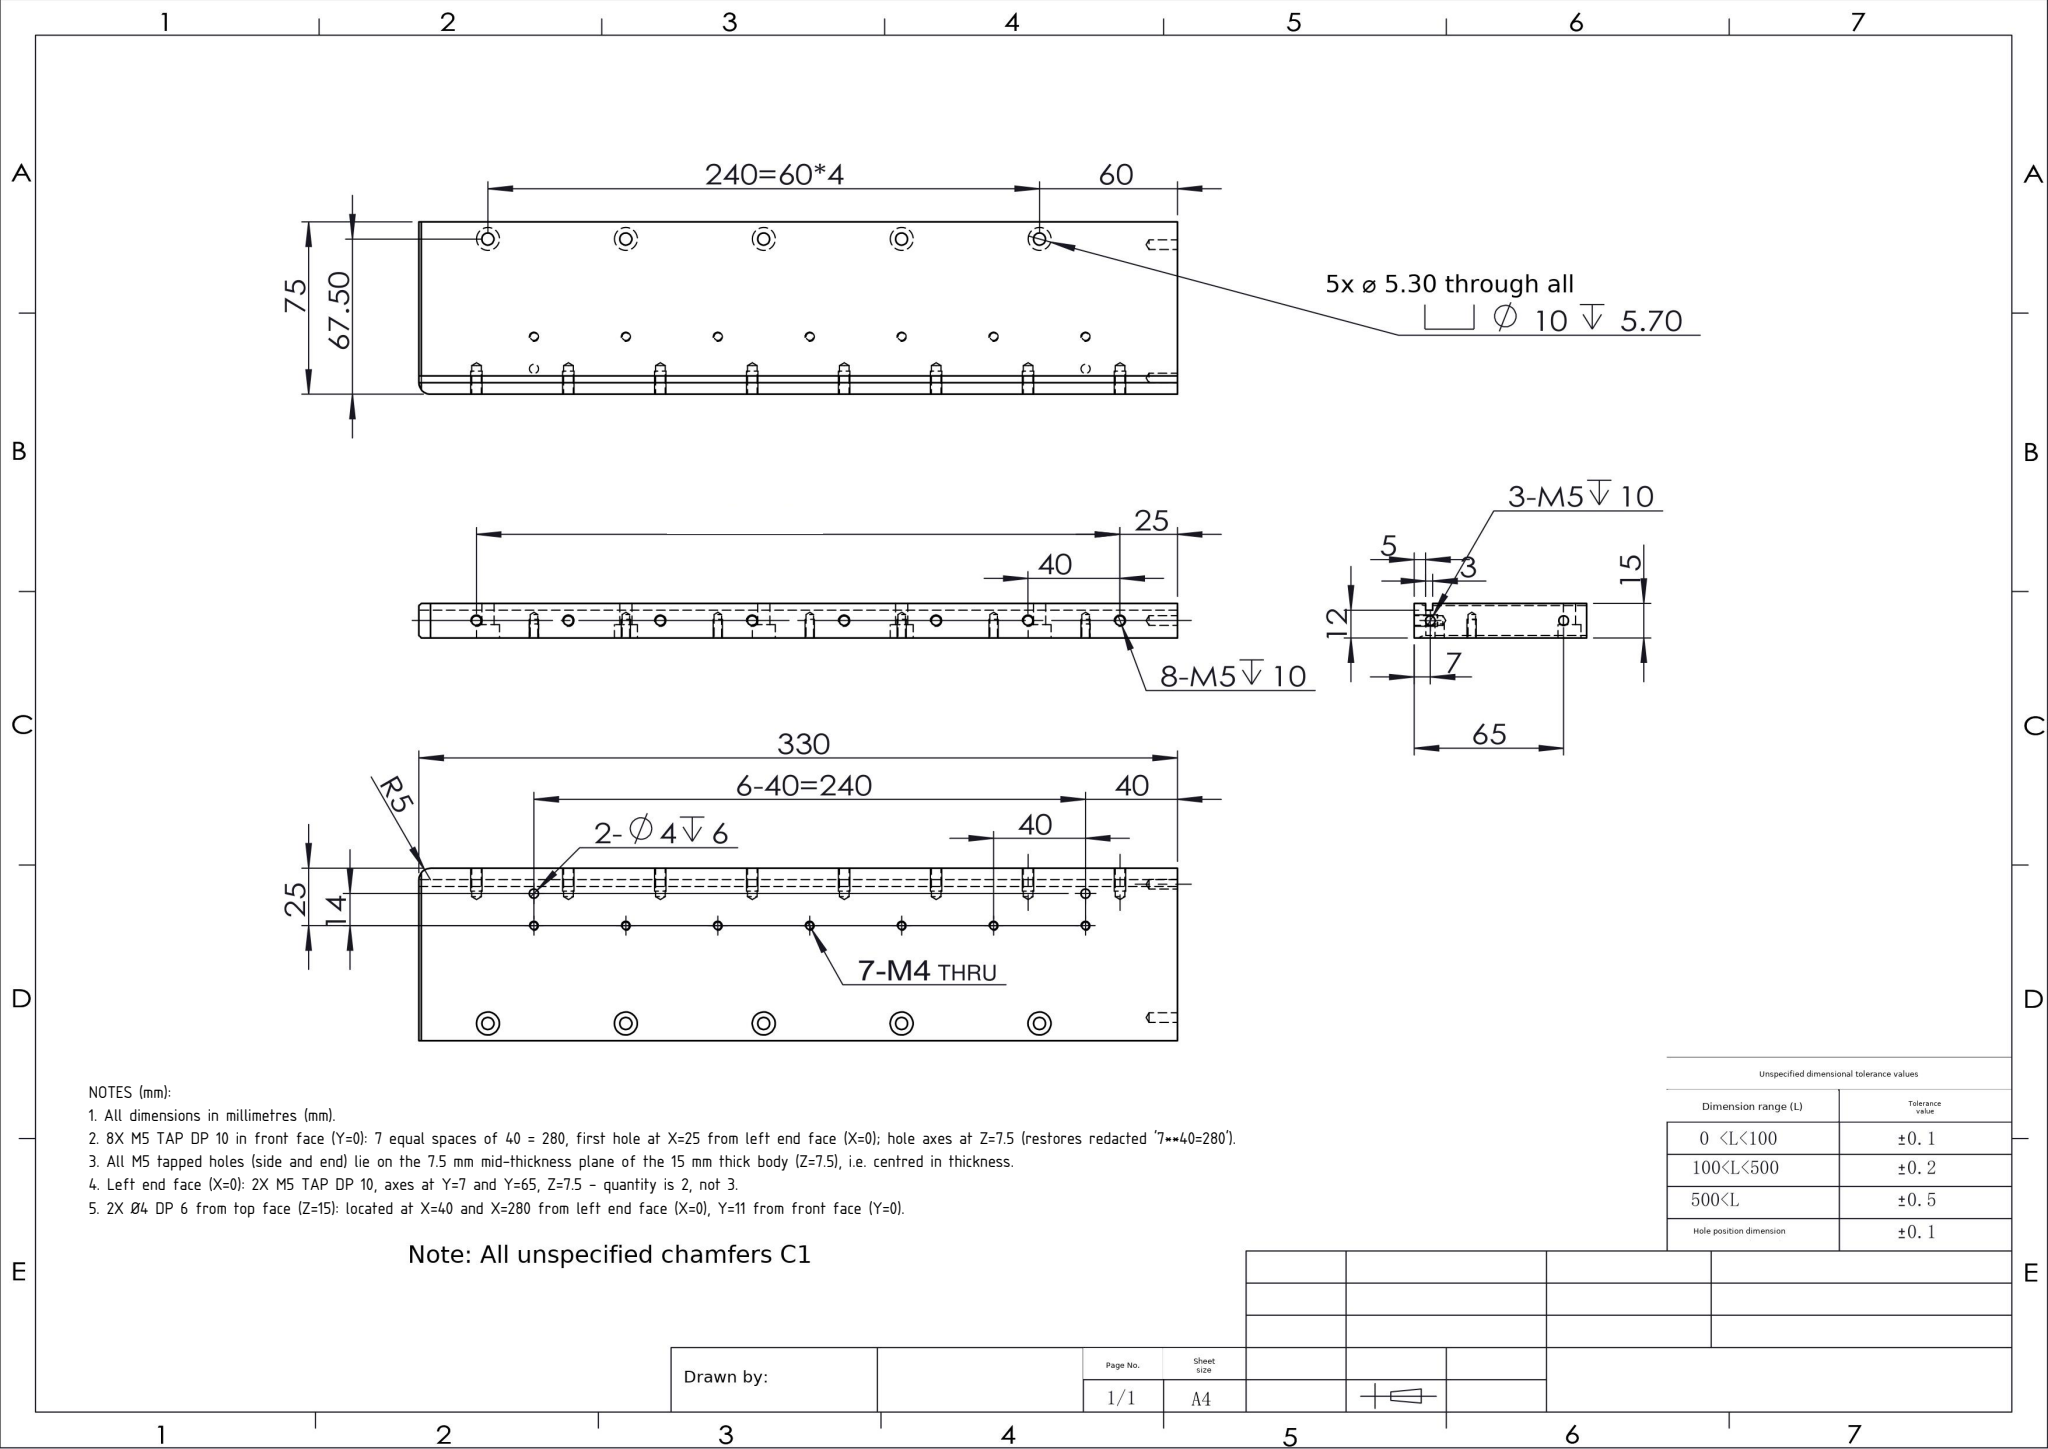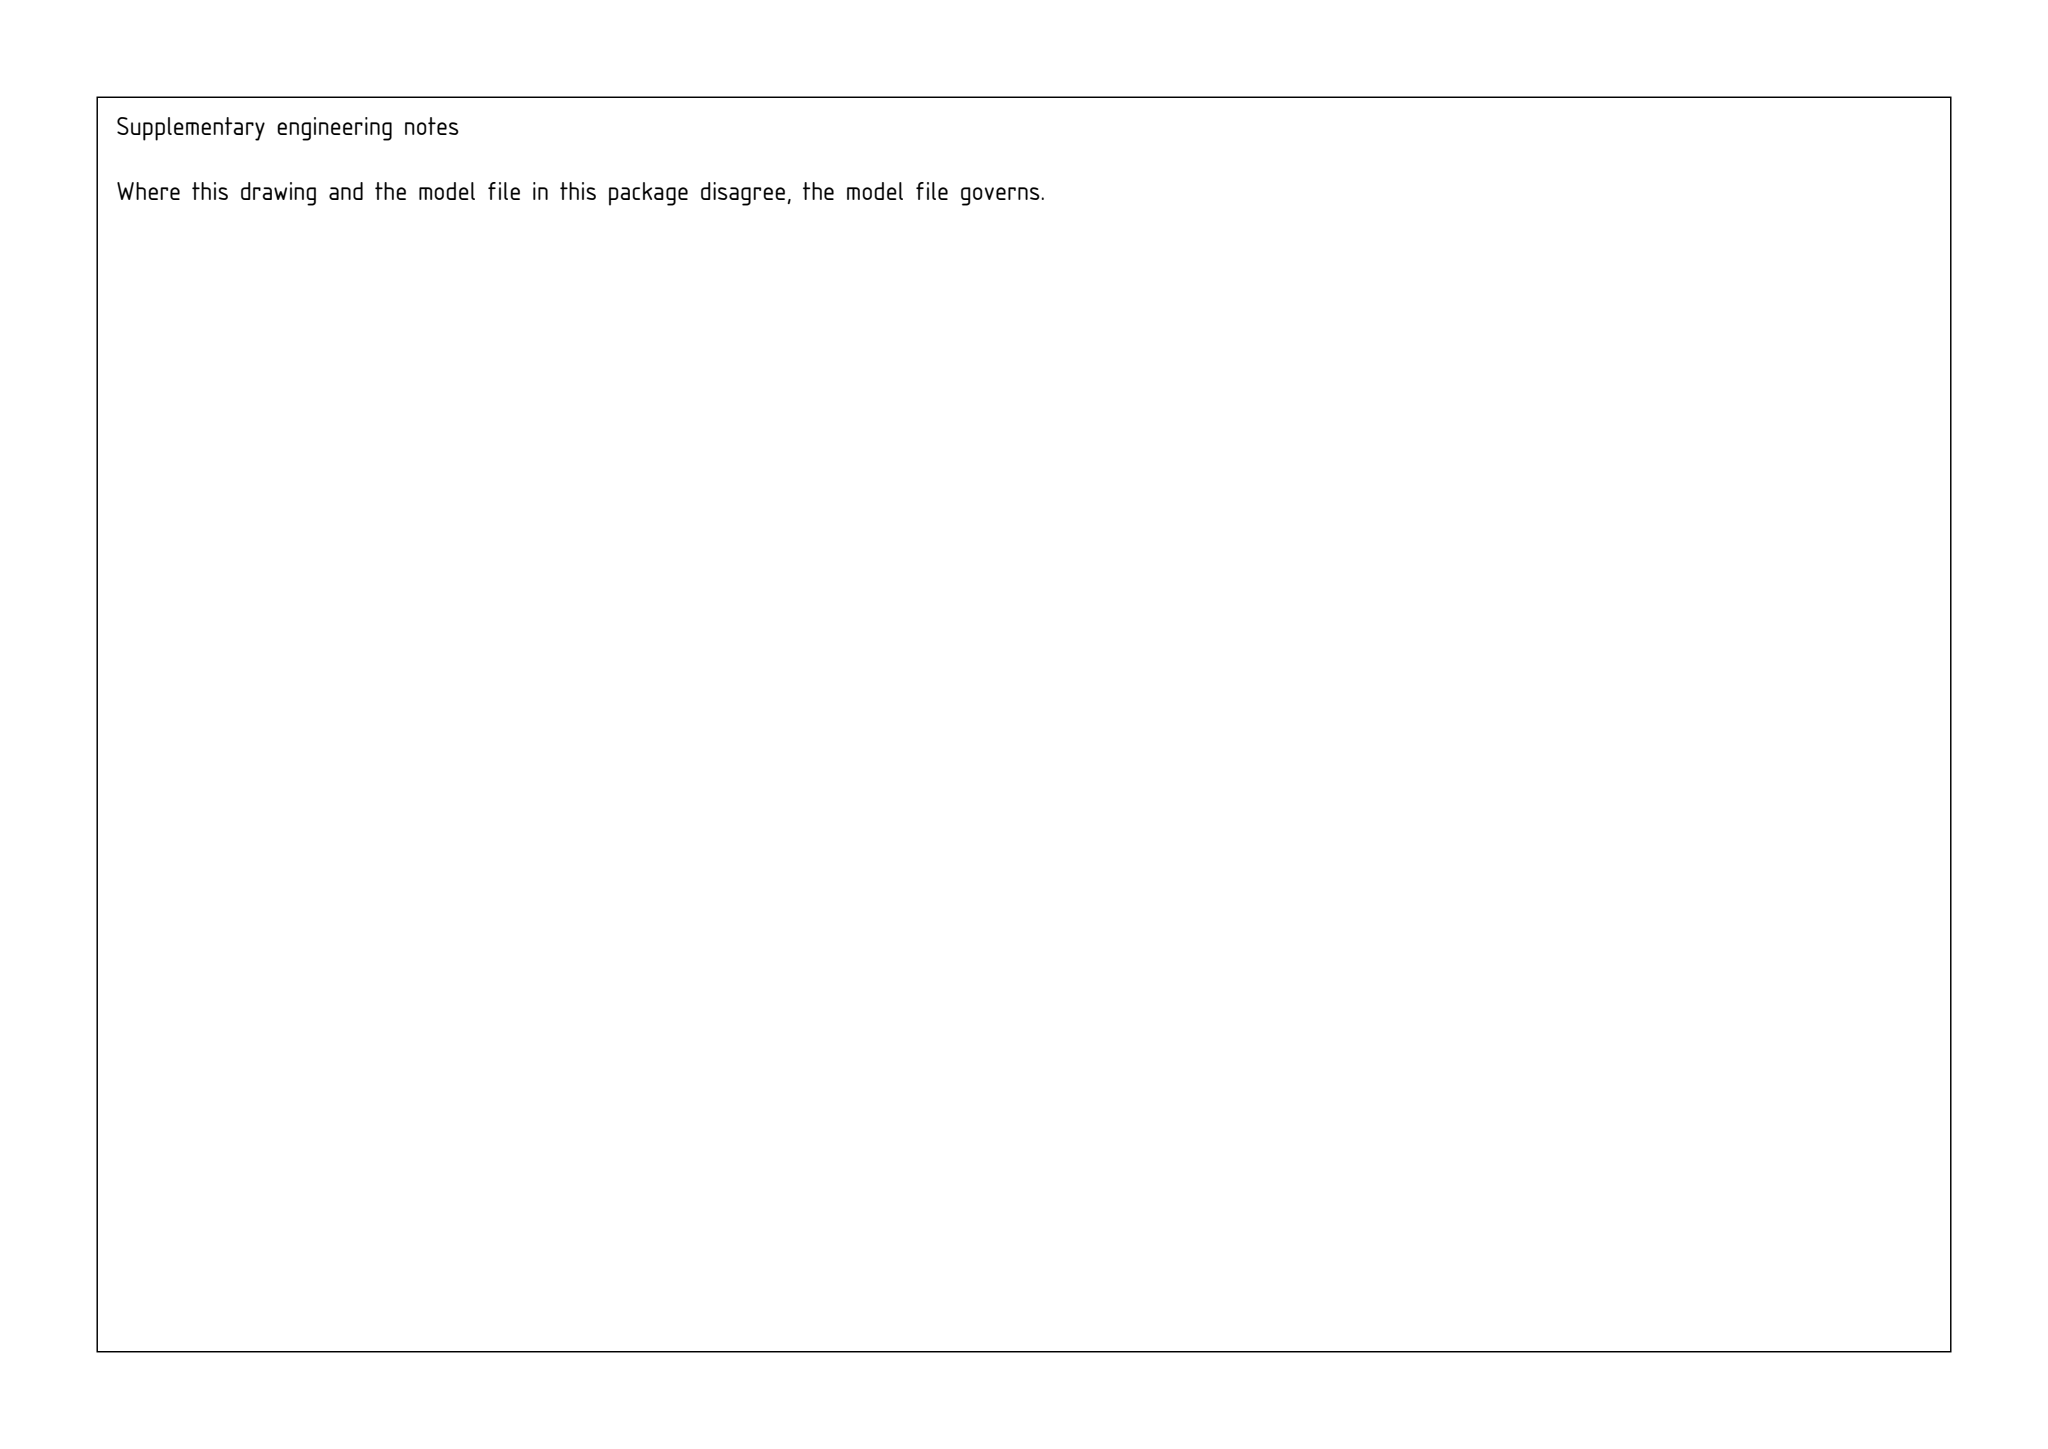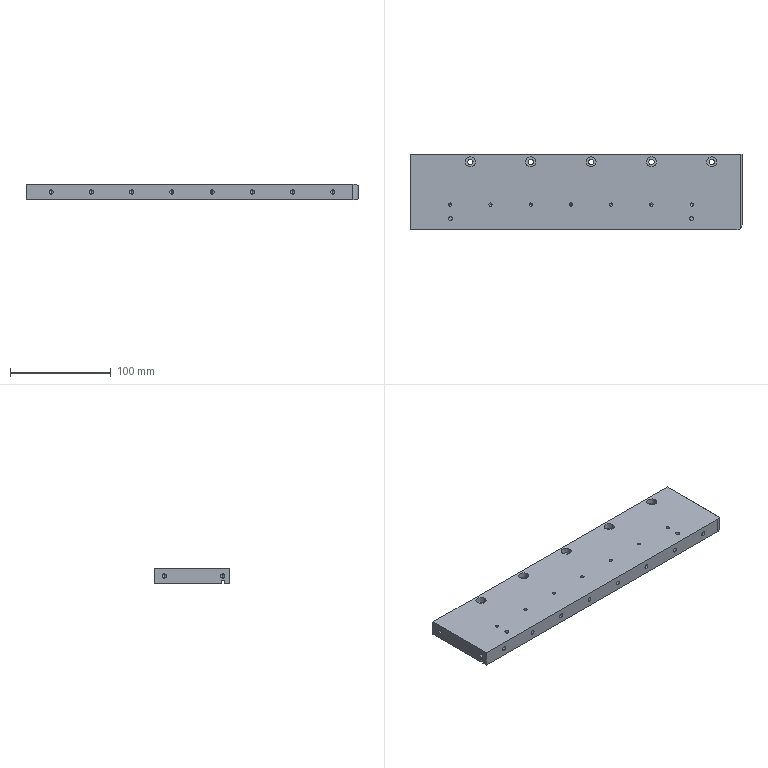Part | SolidWorks | mm | 1 solid | 113 faces | box 330 x 75 x 15 mm | volume 362314 mm3 | cylinder 59 | cone 34 | plane 20 | commonest cylinder face diameters 4.2 x20 3.3 x14 10 x11 5.3 x10 4 x4
Drawing notes:
All dimensions in millimetres (mm). | from the solid: STEP model facts stated in mm; bbox_xyz = 330.0 x 75.0 x 15.0
8X M5 TAP DP 10 in front face (Y=0): 7 equal spaces of 40 = 280, first hole at X=25 from left end face (X=0); hole axes at Z=7.5 (restores redacted '7**40=280'). | from the solid: cylinders: 8x hole/bore dia 4.2, axis y, at x = 25,65,105,145,185,225,265,305, z = 7.5, from 0 to 12.4
All M5 tapped holes (side and end) lie on the 7.5 mm mid-thickness plane of the 15 mm thick body (Z=7.5), i.e. centred in thickness. | from the solid: cylinders: all dia 4.2 bores (axis x and axis y) have axis_pos z = 7.5; bbox z extent 0-15
Left end face (X=0): 2X M5 TAP DP 10, axes at Y=7 and Y=65, Z=7.5 - quantity is 2, not 3. | from the solid: cylinders: only two dia 4.2 bores with axis x, at [y=7.0, z=7.5] and [y=65.0, z=7.5], from 0 to 12.4
2X Ø4 DP 6 from top face (Z=15): located at X=40 and X=280 from left end face (X=0), Y=11 from front face (Y=0). | from the solid: cylinders: hole/bore dia 4.0, axis z, at [40.0, 11.0] and [280.0, 11.0], from 9.0 to 15.0
build123d program:
from build123d import *

# Parameters (mm, degrees)
SKETCH1_W                                            = 330
SKETCH1_H                                            = 100
BOSS_EXTRUDE1_DEPTH                                  = 15
FILLET1_R                                            = 10
CUT_EXTRUDE2_DEPTH                                   = 0.1
CHAMFER1_SIZE                                        = 1
CHAMFER2_SIZE                                        = 1
CUT_EXTRUDE5_START                                   = -12
SKETCH14_W                                           = 717.936
SKETCH14_H                                           = 3
CUT_EXTRUDE5_DEPTH                                   = 3
FILLET5_R                                            = 5
LPATTERN5_COUNT                                      = 8
LPATTERN5_PITCH                                      = 40
M5_TAPPED_HOLE2_D                                    = 4.2
M5_TAPPED_HOLE2_DEPTH                                = 12.4
M5_TAPPED_HOLE2_TIP                                  = 1.262
HOLE_SIZE_ACCORDING_TO_THE_TYPE_OF_HEXAG_D           = 5.3
HOLE_SIZE_ACCORDING_TO_THE_TYPE_OF_HEXAG_CBORE_D     = 10
HOLE_SIZE_ACCORDING_TO_THE_TYPE_OF_HEXAG_CBORE_DEPTH = 5.7
LPATTERN6_COUNT                                      = 5
LPATTERN6_PITCH                                      = 60
LPATTERN7_COUNT                                      = 7
LPATTERN7_PITCH                                      = 40
SKETCH27_R                                           = 2
CUT_EXTRUDE6_DEPTH                                   = 6
SKETCH28_W                                           = 438.351
SKETCH28_H                                           = 72.886
CUT_EXTRUDE7_DEPTH                                   = 346.145
HOLE_SIZE_ACCORDING_TO_THE_TYPE_OF_H_2_D             = 5.3
HOLE_SIZE_ACCORDING_TO_THE_TYPE_OF_H_2_CBORE_D       = 10
HOLE_SIZE_ACCORDING_TO_THE_TYPE_OF_H_2_CBORE_DEPTH   = 5.7


with BuildPart() as part:
    # Sketch1 → Boss-Extrude1 (new body)
    with BuildSketch(Plane.XY):
        with Locations((165, -50)):
            Rectangle(SKETCH1_W, SKETCH1_H)
    extrude(amount=BOSS_EXTRUDE1_DEPTH)

    # Fillet1
    fillet1_edges = [part.edges().sort_by_distance(p)[0] for p in [
        (330, 0, 7.5),
    ]]
    fillet(fillet1_edges, radius=FILLET1_R)

    # Sketch2 → Cut-Extrude2 (cut)
    with BuildSketch(Plane.XY.offset(15)):
        with BuildLine():
            Line((63.85, -16.145), (63.165, -16.311))
            Line((63.165, -16.311), (63.004, -17.061))
            Line((63.004, -17.061), (62.928, -17.444))
            Line((62.928, -17.444), (62.898, -17.565))
            add(Edge.make_bspline(
                [(62.898, -17.565), (62.895, -17.573), (62.89, -17.588), (62.88, -17.605), (62.869, -17.613), (62.856, -17.615), (62.847, -17.604), (62.842, -17.591), (62.84, -17.571), (62.835, -17.545), (62.833, -17.508), (62.829, -17.48), (62.827, -17.464)],
                knots=[0, 0, 0, 0, 1.227, 2.069, 2.596, 3.064, 3.56, 4.322, 5.03, 6.209, 7.852, 10, 10, 10, 10], degree=3))
            Line((62.827, -17.464), (62.803, -17.253))
            add(Edge.make_bspline(
                [(62.803, -17.253), (62.801, -17.235), (62.798, -17.204), (62.796, -17.163), (62.796, -17.134), (62.797, -17.109), (62.804, -17.086), (62.813, -17.069), (62.818, -17.061)],
                knots=[0, 0, 0, 0, 1.604, 2.861, 3.774, 4.323, 5.132, 6, 6, 6, 6], degree=3))
            Line((62.818, -17.061), (62.843, -17.016))
            add(Edge.make_bspline(
                [(62.843, -17.016), (62.848, -17.004), (62.861, -16.976), (62.878, -16.923), (62.895, -16.856), (62.913, -16.778), (62.93, -16.702), (62.944, -16.64), (62.955, -16.599), (62.962, -16.579), (62.964, -16.573)],
                knots=[0, 0, 0, 0, 0.6797, 1.623, 2.844, 4.336, 5.799, 6.891, 7.631, 8, 8, 8, 8], degree=3))
            Line((62.964, -16.573), (63.482, -14.172))
            Line((63.482, -14.172), (63.552, -14.172))
            Line((63.552, -14.172), (64.041, -16.331))
            Line((64.041, -16.331), (64.101, -16.583))
            add(Edge.make_bspline(
                [(64.101, -16.583), (64.107, -16.611), (64.118, -16.662), (64.135, -16.73), (64.148, -16.781), (64.158, -16.808), (64.162, -16.82)],
                knots=[0, 0, 0, 0, 1.426, 2.558, 3.42, 4, 4, 4, 4], degree=3))
            Line((64.162, -16.82), (64.197, -16.915))
            add(Edge.make_bspline(
                [(64.197, -16.915), (64.201, -16.929), (64.208, -16.954), (64.221, -16.988), (64.233, -17.014), (64.249, -17.036), (64.265, -17.053), (64.276, -17.07), (64.277, -17.086), (64.275, -17.1), (64.273, -17.119), (64.272, -17.142), (64.269, -17.174), (64.268, -17.199), (64.268, -17.213)],
                knots=[0, 0, 0, 0, 1.645, 2.997, 4.066, 4.893, 6.03, 6.671, 7.125, 7.802, 8.339, 9.24, 10.452, 12, 12, 12, 12], degree=3))
            Line((64.268, -17.213), (64.247, -17.439))
            Line((64.247, -17.439), (64.237, -17.524))
            add(Edge.make_bspline(
                [(64.237, -17.524), (64.236, -17.534), (64.236, -17.551), (64.231, -17.574), (64.229, -17.59), (64.223, -17.601), (64.212, -17.607), (64.198, -17.603), (64.187, -17.589), (64.184, -17.577), (64.182, -17.57)],
                knots=[0, 0, 0, 0, 1.663, 2.956, 3.874, 4.465, 5.131, 5.832, 6.736, 8, 8, 8, 8], degree=3))
            Line((64.182, -17.57), (64.147, -17.368))
            Line((64.147, -17.368), (63.85, -16.145))
        make_face()
        with BuildLine():
            Line((63.839, -16.069), (63.517, -14.655))
            Line((63.517, -14.655), (63.19, -16.135))
            add(Edge.make_bspline(
                [(63.19, -16.135), (63.218, -16.13), (63.267, -16.123), (63.336, -16.108), (63.4, -16.09), (63.458, -16.074), (63.505, -16.058), (63.536, -16.047), (63.56, -16.036), (63.572, -16.028), (63.578, -16.024)],
                knots=[0, 0, 0, 0, 1.702, 2.938, 4.141, 5.675, 6.466, 7.109, 7.616, 8, 8, 8, 8], degree=3))
            Line((63.578, -16.024), (63.704, -15.939))
            Line((63.704, -15.939), (63.839, -16.069))
        make_face(mode=Mode.SUBTRACT)
    extrude(amount=-CUT_EXTRUDE2_DEPTH, mode=Mode.SUBTRACT)

    # Chamfer1
    chamfer1_edges = [part.edges().sort_by_distance(p)[0] for p in [
        (330, -55, 15),
        (160, 0, 15),
        (327.071, -2.929, 15),
    ]]
    chamfer(chamfer1_edges, length=CHAMFER1_SIZE)

    # Chamfer2
    chamfer2_edges = [part.edges().sort_by_distance(p)[0] for p in [
        (160, 0, 0),
        (327.071, -2.929, 0),
        (330, -55, 0),
    ]]
    chamfer(chamfer2_edges, length=CHAMFER2_SIZE)

    # Sketch14 → Cut-Extrude5 (cut)
    with BuildSketch(Plane.XY.offset(15).offset(CUT_EXTRUDE5_START)):
        with Locations((338.968, -93.5)):
            Rectangle(SKETCH14_W, SKETCH14_H)
    extrude(amount=-CUT_EXTRUDE5_DEPTH, mode=Mode.SUBTRACT)

    # Fillet5
    fillet5_edges = [part.edges().sort_by_distance(p)[0] for p in [
        (330, -100, 7.5),
    ]]
    fillet(fillet5_edges, radius=FILLET5_R)

    # Sketch19 → M5 Tapped Hole1 (revolve, cut)
    with BuildSketch(Plane(origin=(25, -100, 7.5), x_dir=(0, 0, -1), z_dir=(1, 0, 0))):
        Polygon((0, 0), (0, 13.662), (2.1, 12.4), (2.1, 0), align=None)
    m5_tapped_hole1 = revolve(axis=Axis((25, -106.35, 7.5), (0, 1, 0)), mode=Mode.SUBTRACT)

    # LPattern5: M5 Tapped Hole1 ×8
    with Locations(*[(i * LPATTERN5_PITCH, 0, 0) for i in range(1, LPATTERN5_COUNT)]):
        add(m5_tapped_hole1, mode=Mode.SUBTRACT)

    # M5 Tapped Hole2
    with Locations(Plane.ZY):
        with Locations((7.5, -35), (7.5, -93)):
            Hole(M5_TAPPED_HOLE2_D / 2, depth=M5_TAPPED_HOLE2_DEPTH)
            with Locations((0, 0, -(M5_TAPPED_HOLE2_DEPTH + M5_TAPPED_HOLE2_TIP / 2))):  # 118° drill point
                Cone(0, M5_TAPPED_HOLE2_D / 2, M5_TAPPED_HOLE2_TIP, mode=Mode.SUBTRACT)

    # Hole Size according to the type of hexag (through all)
    with Locations(Plane(origin=(0, 0, 0), x_dir=(-1, 0, 0), z_dir=(0, 0, -1))):
        with Locations((-60, -20)):
            hole_size_according_to_the_type_of_hexag = CounterBoreHole(HOLE_SIZE_ACCORDING_TO_THE_TYPE_OF_HEXAG_D / 2, HOLE_SIZE_ACCORDING_TO_THE_TYPE_OF_HEXAG_CBORE_D / 2, HOLE_SIZE_ACCORDING_TO_THE_TYPE_OF_HEXAG_CBORE_DEPTH)

    # LPattern6: Hole Size according to the type of hexag ×5
    with Locations(*[(i * LPATTERN6_PITCH, 0, 0) for i in range(1, LPATTERN6_COUNT)]):
        add(hole_size_according_to_the_type_of_hexag, mode=Mode.SUBTRACT)

    # Sketch25 → M4 Tapped Hole1 (revolve, cut)
    with BuildSketch(Plane(origin=(40, -75, 15), x_dir=(0, -1, 0), z_dir=(1, 0, 0))):
        Polygon((0, 0), (0, 11.091), (1.65, 10.1), (1.65, 0), align=None)
    m4_tapped_hole1 = revolve(axis=Axis((40, -75, 21.35), (0, 0, -1)), mode=Mode.SUBTRACT)

    # LPattern7: M4 Tapped Hole1 ×7
    with Locations(*[(i * LPATTERN7_PITCH, 0, 0) for i in range(1, LPATTERN7_COUNT)]):
        add(m4_tapped_hole1, mode=Mode.SUBTRACT)

    # Sketch27 → Cut-Extrude6 (cut)
    with BuildSketch(Plane.XY.offset(15)):
        with Locations((40, -89)):
            Circle(SKETCH27_R)
        with Locations((280, -89)):
            Circle(SKETCH27_R)
    extrude(amount=-CUT_EXTRUDE6_DEPTH, mode=Mode.SUBTRACT)

    # Sketch28 → Cut-Extrude7 (cut, through all)
    with BuildSketch(Plane.XY.offset(15)):
        with Locations((153.693, 11.443)):
            Rectangle(SKETCH28_W, SKETCH28_H)
    extrude(amount=-CUT_EXTRUDE7_DEPTH, mode=Mode.SUBTRACT)

    # Hole Size according to the type of h 2 (through all)
    with Locations(Plane.XY.offset(15)):
        with Locations((60, -32.5), (120, -32.5), (180, -32.5), (240, -32.5), (300, -32.5)):
            CounterBoreHole(HOLE_SIZE_ACCORDING_TO_THE_TYPE_OF_H_2_D / 2, HOLE_SIZE_ACCORDING_TO_THE_TYPE_OF_H_2_CBORE_D / 2, HOLE_SIZE_ACCORDING_TO_THE_TYPE_OF_H_2_CBORE_DEPTH)


solid = part.part